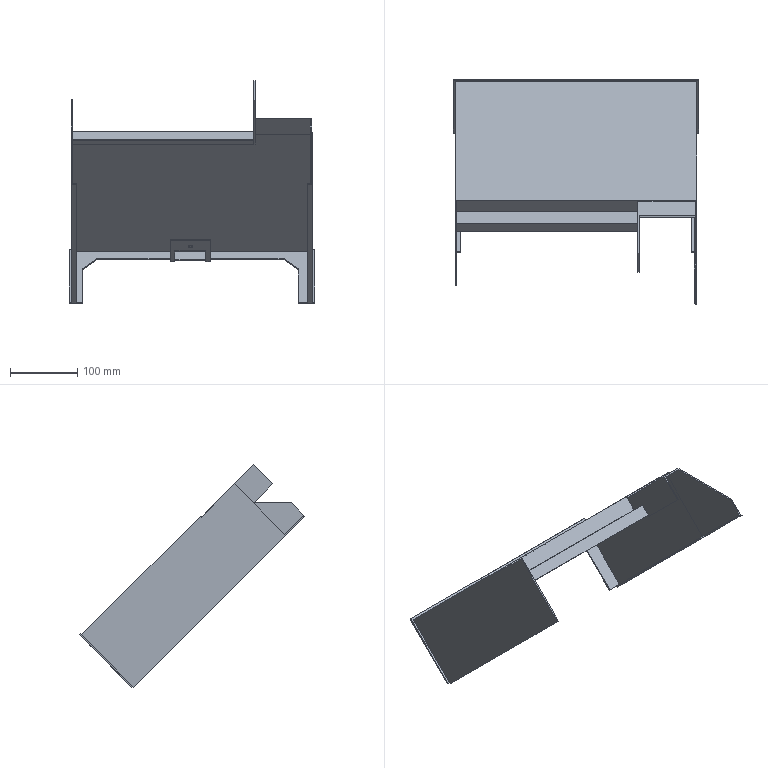Component | SolidWorks | GeneralAssembly-1_1-1 | 3 solids | 64 faces | box 366 x 335.88 x 330.93 mm | volume 412579 mm3 | plane 62 | cylinder 2 | commonest cylinder face diameters 6 x2
build123d program:
from build123d import *

# Parameters (mm, degrees)
EXTRUDE_THIN1_DEPTH = 250
SKETCH2_W           = 272
SKETCH2_H           = 25
BOSS_EXTRUDE1_DEPTH = 2
SKETCH3_W           = 270
SKETCH3_H           = 2
EXTRUDE_THIN2_DEPTH = 25
SKETCH4_W           = 270
SKETCH4_H           = 17
BOSS_EXTRUDE2_DEPTH = 2
SKETCH5_W           = 2
SKETCH5_H           = 80
BOSS_EXTRUDE3_DEPTH = 70
BOSS_EXTRUDE5_DEPTH = 2
EXTRUDE_THIN4_DEPTH = 110
CUT_EXTRUDE3_DEPTH  = 84
CUT_EXTRUDE2_DEPTH  = 2
SKETCH12_W          = 70
SKETCH12_H          = 28
BOSS_EXTRUDE6_DEPTH = 2
BOSS_EXTRUDE7_DEPTH = 2
SKETCH16_W          = 60
SKETCH16_H          = 45
BOSS_EXTRUDE8_DEPTH = 4
SKETCH17_W          = 46
SKETCH17_H          = 23
CUT_EXTRUDE4_DEPTH  = 2
SKETCH18_W          = 43
SKETCH18_H          = 2
CUT_EXTRUDE5_DEPTH  = 60
SKETCH19_R          = 3
CUT_EXTRUDE6_DEPTH  = 2


with BuildPart() as part:
    # Sketch1 → Extrude-Thin1 (new body)
    with BuildSketch(Plane.XY):
        Polygon((-38.343, -96.506), (-46.343, -96.506), (-46.343, 13.494), (313.657, 13.494), (313.657, -96.506), (305.657, -96.506), (305.657, -94.506), (311.657, -94.506), (311.657, 11.494), (-44.343, 11.494), (-44.343, -94.506), (-38.343, -94.506), align=None)
    extrude(amount=EXTRUDE_THIN1_DEPTH)

    # Sketch2 → Boss-Extrude1 (add)
    with BuildSketch(Plane.XY.offset(250)):
        with Locations((89.657, 0.9938)):
            Rectangle(SKETCH2_W, SKETCH2_H)
    extrude(amount=-BOSS_EXTRUDE1_DEPTH)

    # Sketch3 → Extrude-Thin2 (add)
    with BuildSketch(Plane.XY.offset(250)):
        with Locations((90.657, -10.506)):
            Rectangle(SKETCH3_W, SKETCH3_H)
    extrude(amount=EXTRUDE_THIN2_DEPTH)

    # Sketch4 → Boss-Extrude2 (add)
    with BuildSketch(Plane.XY.offset(275)):
        with Locations((90.657, -18.006)):
            Rectangle(SKETCH4_W, SKETCH4_H)
    extrude(amount=-BOSS_EXTRUDE2_DEPTH)

    # Sketch5 → Boss-Extrude3 (add)
    with BuildSketch(Plane.XY.offset(250)):
        with Locations((-45.343, -28.506)):
            Rectangle(SKETCH5_W, SKETCH5_H)
    extrude(amount=BOSS_EXTRUDE3_DEPTH)

    # Sketch11 → Boss-Extrude5 (add)
    with BuildSketch(Plane(origin=(313.657, 0, 0), x_dir=(0, 0, -1), z_dir=(1, 0, 0))):
        Polygon((-250, 13.494), (-360, -96.506), (-250, -96.506), align=None)
    extrude(amount=-BOSS_EXTRUDE5_DEPTH)

    # Sketch12 → Boss-Extrude6 (add)
    with BuildSketch(Plane.ZY.offset(46.343)):
        with Locations((285, -82.506)):
            Rectangle(SKETCH12_W, SKETCH12_H)
    extrude(amount=-BOSS_EXTRUDE6_DEPTH)


with BuildPart() as body_2:
    # Sketch6 → Extrude-Thin4 (new body)
    with BuildSketch(Plane.XY.offset(250)):
        Polygon((225.657, -32.767), (225.657, 11.494), (311.657, 11.494), (311.657, -94.506), (309.657, -94.506), (309.657, 9.494), (227.657, 9.494), (227.657, -32.767), align=None)
    extrude(amount=EXTRUDE_THIN4_DEPTH)

    # Sketch14 → Cut-Extrude3 (cut)
    with BuildSketch(Plane(origin=(311.657, 0, 0), x_dir=(0, 0, -1), z_dir=(1, 0, 0))):
        Polygon((-360, 11.494), (-280.284, 11.494), (-360, -68.222), align=None)
    extrude(amount=-CUT_EXTRUDE3_DEPTH, mode=Mode.SUBTRACT)

    # Sketch9 → Cut-Extrude2 (cut)
    with BuildSketch(Plane.ZY.offset(-225.657)):
        Polygon((250, -11.506), (273, -11.506), (273, -28.767), (360, -28.767), (360, -32.767), (250, -32.767), align=None)
    extrude(amount=-CUT_EXTRUDE2_DEPTH, mode=Mode.SUBTRACT)


with BuildPart() as body_3:
    # Sketch15 → Boss-Extrude7 (new body)
    with BuildSketch(Plane(origin=(0, 0, 0), x_dir=(-1, 0, 0), z_dir=(0, 0, -1))):
        Polygon((-291.657, -94.506), (-311.657, -94.506), (-316.657, -94.506), (-316.657, 16.494), (49.343, 16.494), (49.343, -94.506), (29.343, -94.506), (29.343, -24.506), (8.343, -3.506), (-270.657, -3.506), (-291.657, -24.506), align=None)
    extrude(amount=BOSS_EXTRUDE7_DEPTH)

    # Sketch16 → Boss-Extrude8 (add)
    with BuildSketch(Plane.XZ.offset(3.506)):
        with Locations((131.157, 20.5)):
            Rectangle(SKETCH16_W, SKETCH16_H)
    extrude(amount=BOSS_EXTRUDE8_DEPTH)

    # Sketch17 → Cut-Extrude4 (cut)
    with BuildSketch(Plane.XZ.offset(7.506)):
        with Locations((131.157, 9.5)):
            Rectangle(SKETCH17_W, SKETCH17_H)
    extrude(amount=-CUT_EXTRUDE4_DEPTH, mode=Mode.SUBTRACT)

    # Sketch18 → Cut-Extrude5 (cut)
    with BuildSketch(Plane.ZY.offset(-101.157)):
        with Locations((21.5, -4.506)):
            Rectangle(SKETCH18_W, SKETCH18_H)
    extrude(amount=-CUT_EXTRUDE5_DEPTH, mode=Mode.SUBTRACT)

    # Sketch19 → Cut-Extrude6 (cut)
    with BuildSketch(Plane(origin=(0, -7.506, 0), x_dir=(-1, 0, 0), z_dir=(0, -1, 0))):
        with Locations(Location((-131.157, -30.14, 0), (0, 0, 180))):
            Circle(SKETCH19_R)
    extrude(amount=-CUT_EXTRUDE6_DEPTH, mode=Mode.SUBTRACT)


solid = Compound([part.part, body_2.part, body_3.part])

# Placed as in the assembly
solid = solid.moved(Location((28.168, 395.972, -521.739), (45, 0, 0)))